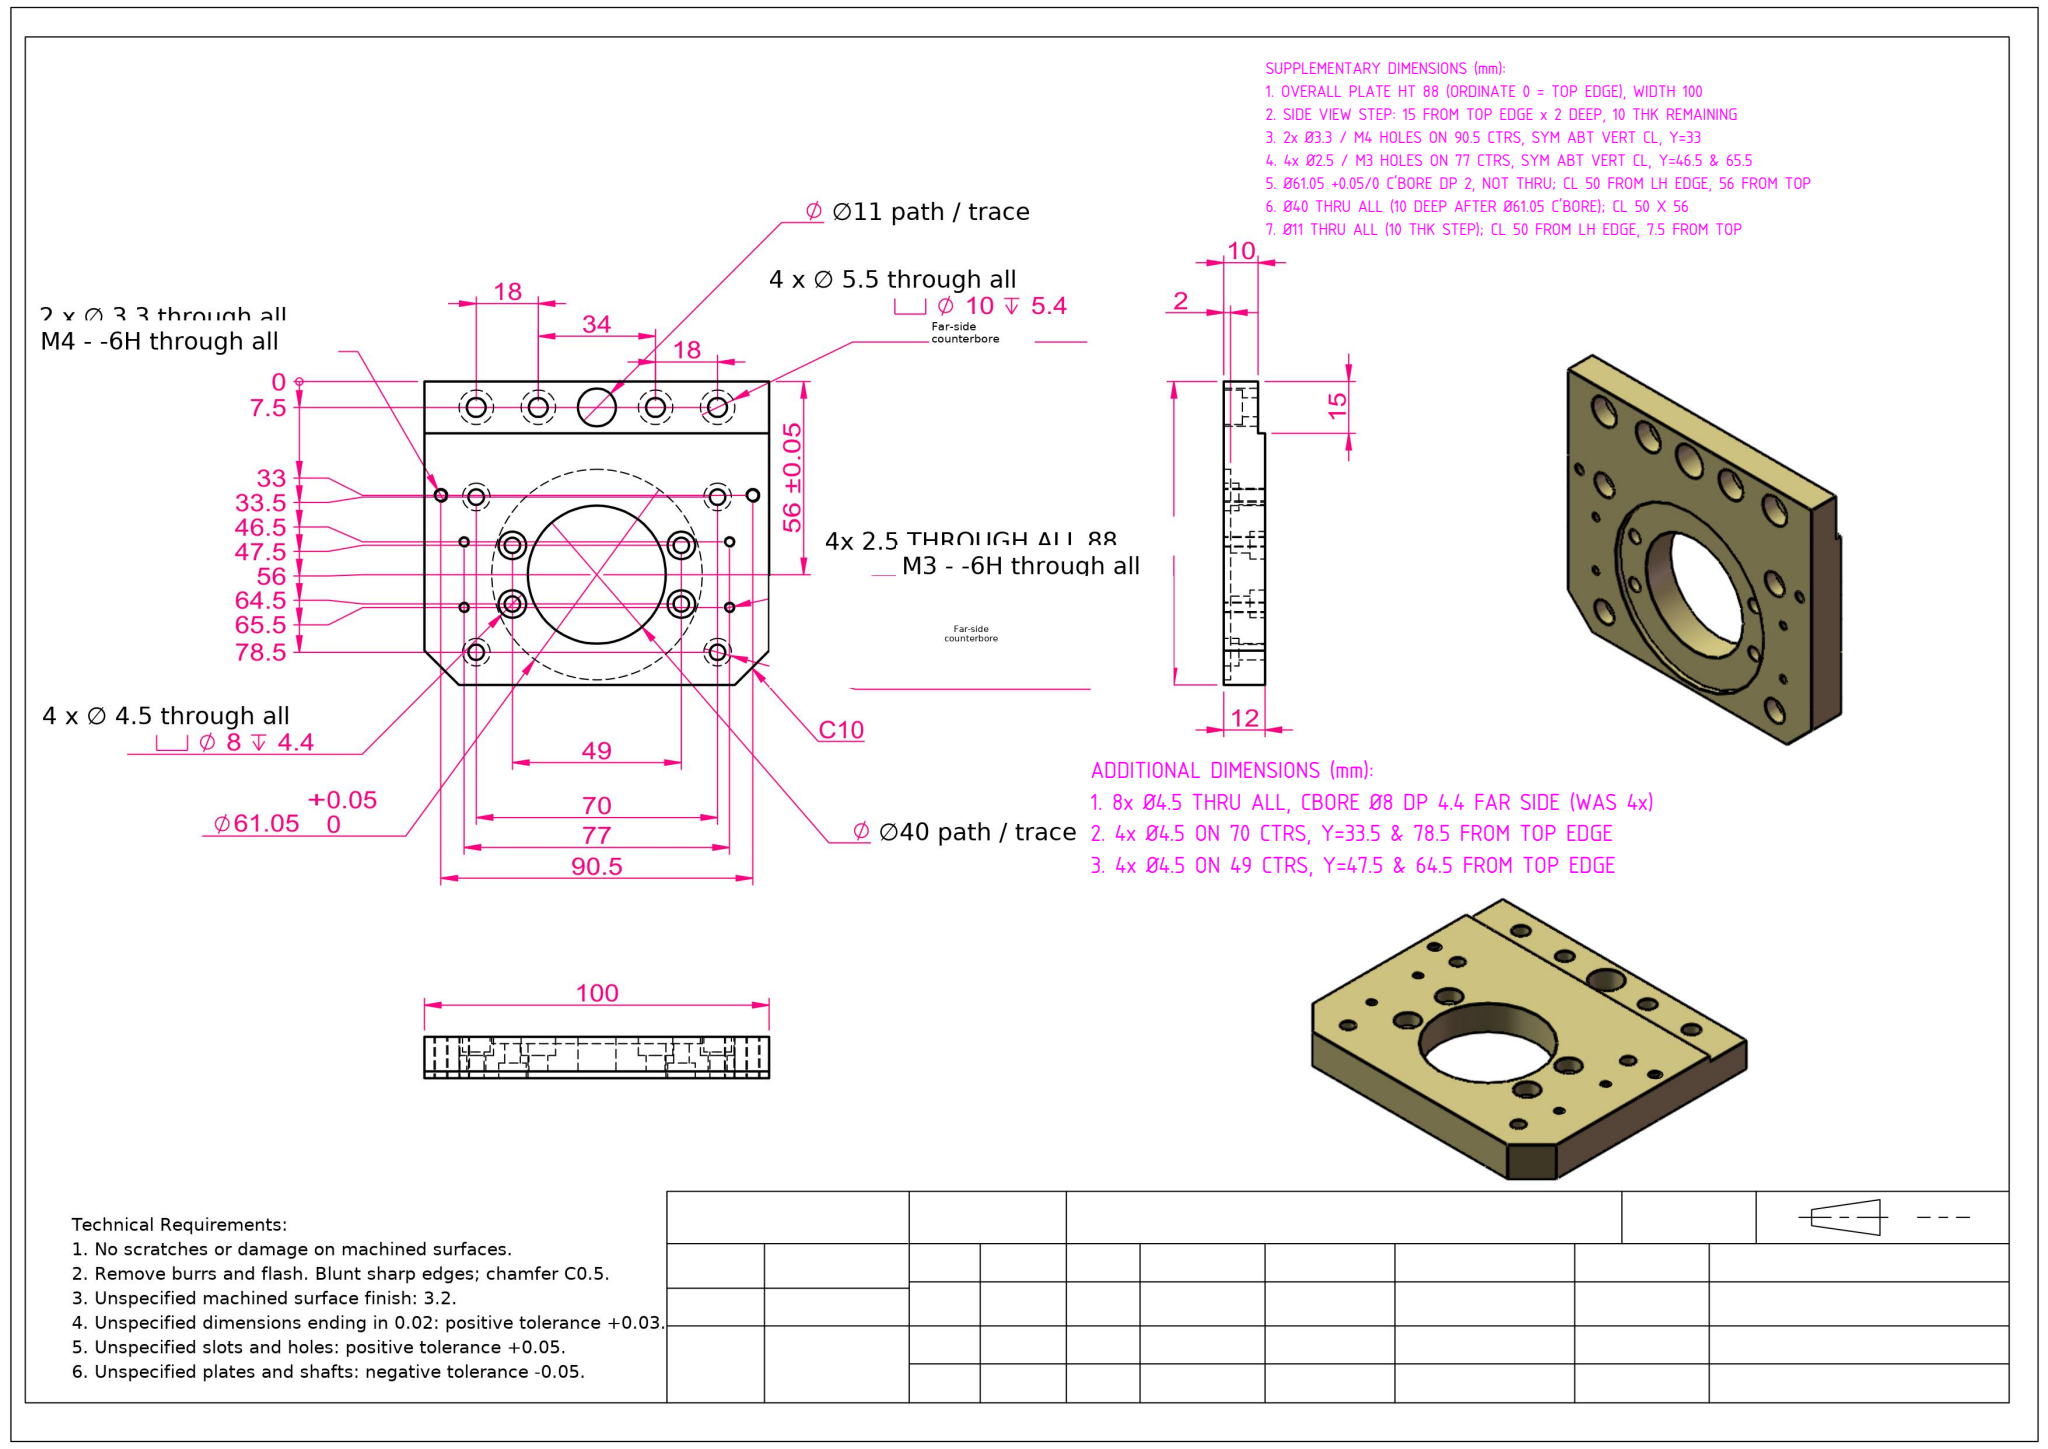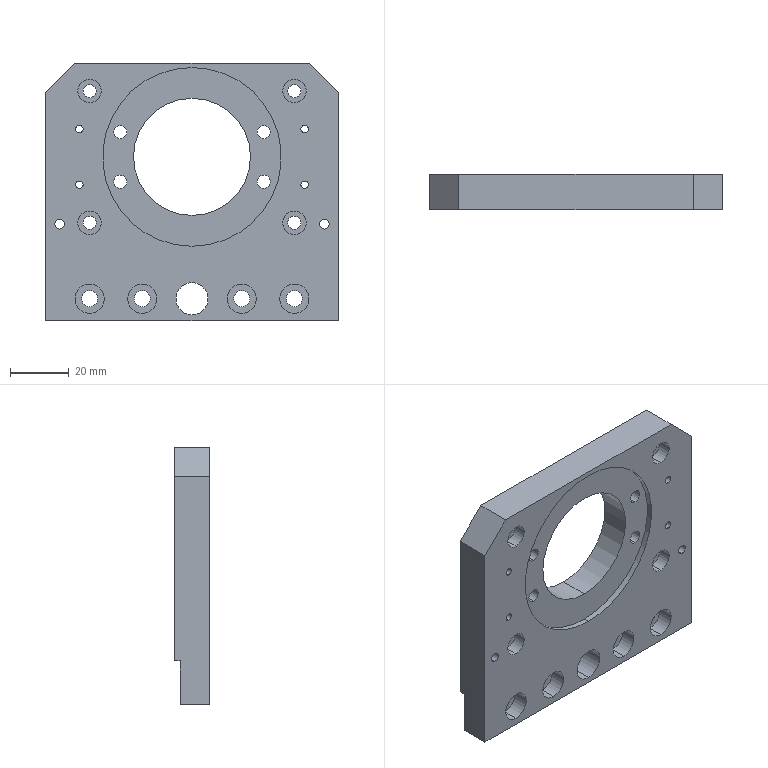Part | SolidWorks | mm | 1 solid | 89 faces | box 100 x 12 x 88 mm | volume 76845 mm3 | cylinder 66 | plane 23 | commonest cylinder face diameters 8 x16 4.5 x16 2.5 x8 10 x8 5.5 x8 3.3 x4 61.05 x2 11 x2
build123d program:
from build123d import *

# Parameters (mm, degrees)
SKETCH1_W                                       = 100
SKETCH1_H                                       = 88
BOSS_EXTRUDE1_DEPTH                             = 12
SKETCH2_R                                       = 20
CUT_EXTRUDE1_DEPTH                              = 68.676
SKETCH3_W                                       = 100
SKETCH3_H                                       = 15
CUT_EXTRUDE2_DEPTH                              = 2
M5_HEX_SOCKET_HEAD_CAP_SCREW_CBORE1_D           = 5.5
M5_HEX_SOCKET_HEAD_CAP_SCREW_CBORE1_CBORE_D     = 10
M5_HEX_SOCKET_HEAD_CAP_SCREW_CBORE1_CBORE_DEPTH = 5.4
SKETCH6_R                                       = 5.5
CUT_EXTRUDE3_DEPTH                              = 68.676
CHAMFER1_SIZE                                   = 10
M4_HEX_SOCKET_HEAD_CAP_SCREW_CBORE1_D           = 4.5
M4_HEX_SOCKET_HEAD_CAP_SCREW_CBORE1_CBORE_D     = 8
M4_HEX_SOCKET_HEAD_CAP_SCREW_CBORE1_CBORE_DEPTH = 4.4
M4_HEX_SOCKET_HEAD_CAP_SCREW_CBORE2_D           = 4.5
M4_HEX_SOCKET_HEAD_CAP_SCREW_CBORE2_CBORE_D     = 8
M4_HEX_SOCKET_HEAD_CAP_SCREW_CBORE2_CBORE_DEPTH = 4.4
SKETCH21_R                                      = 30.525
CUT_EXTRUDE4_DEPTH                              = 2
M3_TAPPED_HOLE2_D                               = 2.5
M4_TAPPED_HOLE2_D                               = 3.3


with BuildPart() as part:
    # Sketch1 → Boss-Extrude1 (new body)
    with BuildSketch(Plane(origin=(0, 26, 0), x_dir=(1, 0, 0), z_dir=(0, 1, 0))):
        Rectangle(SKETCH1_W, SKETCH1_H)
    extrude(amount=-BOSS_EXTRUDE1_DEPTH)

    # Sketch2 → Cut-Extrude1 (cut, through all)
    with BuildSketch(Plane(origin=(0, 26, 0), x_dir=(1, 0, 0), z_dir=(0, 1, 0))):
        with Locations(Location((0, -12, 0), (0, 0, 270))):
            Circle(SKETCH2_R)
    extrude(amount=-CUT_EXTRUDE1_DEPTH, mode=Mode.SUBTRACT)

    # Sketch3 → Cut-Extrude2 (cut)
    with BuildSketch(Plane(origin=(0, 26, 0), x_dir=(1, 0, 0), z_dir=(0, 1, 0))):
        with Locations((0, 36.5)):
            Rectangle(SKETCH3_W, SKETCH3_H)
    extrude(amount=-CUT_EXTRUDE2_DEPTH, mode=Mode.SUBTRACT)

    # M5 Hex Socket Head Cap Screw CBORE1 (through all)
    with Locations(Plane(origin=(0, 14, 0), x_dir=(-1, 0, 0), z_dir=(0, -1, 0))):
        with Locations((35, 36.5), (17, 36.5), (-17, 36.5), (-35, 36.5)):
            CounterBoreHole(M5_HEX_SOCKET_HEAD_CAP_SCREW_CBORE1_D / 2, M5_HEX_SOCKET_HEAD_CAP_SCREW_CBORE1_CBORE_D / 2, M5_HEX_SOCKET_HEAD_CAP_SCREW_CBORE1_CBORE_DEPTH)

    # Sketch6 → Cut-Extrude3 (cut, through all)
    with BuildSketch(Plane.XZ.offset(-14)):
        with Locations(Location((0, -36.5, 0), (0, 0, 270))):
            Circle(SKETCH6_R)
    extrude(amount=-CUT_EXTRUDE3_DEPTH, mode=Mode.SUBTRACT)

    # Chamfer1
    chamfer1_edges = [part.edges().sort_by_distance(p)[0] for p in [
        (50, 20, 44),
        (-50, 20, 44),
    ]]
    chamfer(chamfer1_edges, length=CHAMFER1_SIZE)

    # M4 Hex Socket Head Cap Screw CBORE1 (through all)
    with Locations(Plane(origin=(0, 26, 0), x_dir=(1, 0, 0), z_dir=(0, 1, 0))):
        with Locations((-24.5, -3.5), (-24.5, -20.5), (24.5, -20.5), (24.5, -3.5)):
            CounterBoreHole(M4_HEX_SOCKET_HEAD_CAP_SCREW_CBORE1_D / 2, M4_HEX_SOCKET_HEAD_CAP_SCREW_CBORE1_CBORE_D / 2, M4_HEX_SOCKET_HEAD_CAP_SCREW_CBORE1_CBORE_DEPTH)

    # M4 Hex Socket Head Cap Screw CBORE2 (through all)
    with Locations(Plane(origin=(0, 14, 0), x_dir=(-1, 0, 0), z_dir=(0, -1, 0))):
        with Locations((35, 10.5), (-35, 10.5), (35, -34.5), (-35, -34.5)):
            CounterBoreHole(M4_HEX_SOCKET_HEAD_CAP_SCREW_CBORE2_D / 2, M4_HEX_SOCKET_HEAD_CAP_SCREW_CBORE2_CBORE_D / 2, M4_HEX_SOCKET_HEAD_CAP_SCREW_CBORE2_CBORE_DEPTH)

    # Sketch21 → Cut-Extrude4 (cut)
    with BuildSketch(Plane.XZ.offset(-14)):
        with Locations(Location((0, 12, 0), (0, 0, 270))):
            Circle(SKETCH21_R)
    extrude(amount=-CUT_EXTRUDE4_DEPTH, mode=Mode.SUBTRACT)

    # M3 Tapped Hole2 (through all)
    with Locations(Plane(origin=(0, 26, 0), x_dir=(1, 0, 0), z_dir=(0, 1, 0))):
        with Locations((-38.5, -21.5), (-38.5, -2.5), (38.5, -2.5), (38.5, -21.5)):
            Hole(M3_TAPPED_HOLE2_D / 2)

    # M4 Tapped Hole2 (through all)
    with Locations(Plane(origin=(0, 26, 0), x_dir=(1, 0, 0), z_dir=(0, 1, 0))):
        with Locations((-45.25, 11), (45.25, 11)):
            Hole(M4_TAPPED_HOLE2_D / 2)


solid = part.part